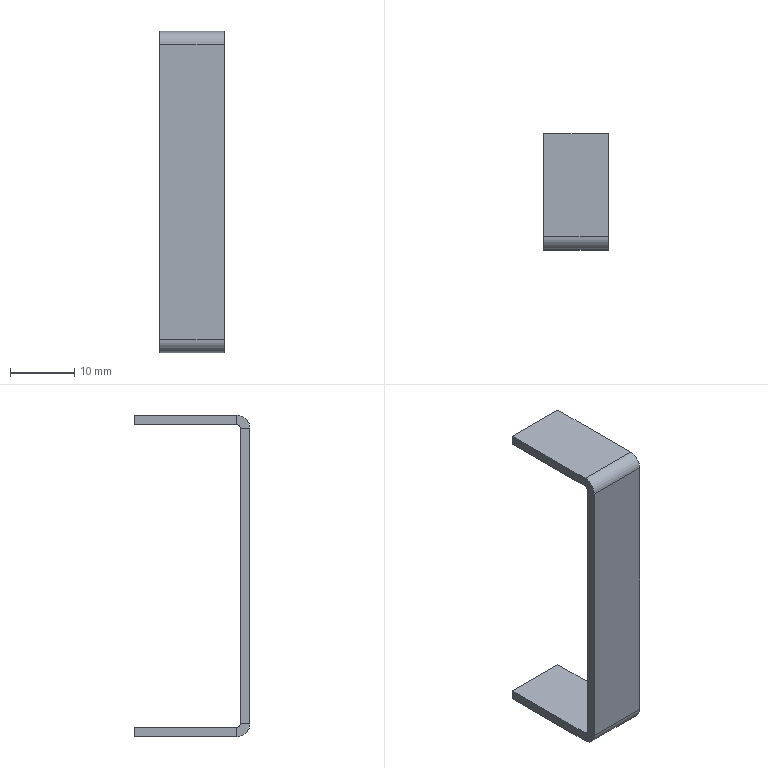Component | SolidWorks | OuterDoorAssembly1-1_CableSupportBracket-1 | 1 solid | 22 faces | box 10.01 x 18 x 50 mm | volume 1229 mm3 | plane 18 | cylinder 4 | commonest cylinder face diameters 4 x2 1 x2
STEP:
#1=CARTESIAN_POINT('',(17.943,6.43,12.714));
#2=VERTEX_POINT('',#1);
#3=CARTESIAN_POINT('',(17.943,6.489,12.714));
#4=VERTEX_POINT('',#3);
#5=CARTESIAN_POINT('',(17.943,6.43,12.714));
#6=DIRECTION('',(0.0003491,1.,-0.));
#7=VECTOR('',#6,39.37);
#8=LINE('',#5,#7);
#9=EDGE_CURVE('',#2,#4,#8,.T.);
#10=ORIENTED_EDGE('',*,*,#9,.F.);
#11=CARTESIAN_POINT('',(17.943,6.509,12.793));
#12=VERTEX_POINT('',#11);
#13=CARTESIAN_POINT('',(17.943,6.509,12.714));
#14=DIRECTION('',(1.,-0.0003491,0.));
#15=DIRECTION('',(-0.0003491,-1.,0.));
#16=AXIS2_PLACEMENT_3D('',#13,#14,#15);
#17=CIRCLE('',#16,0.07874);
#18=EDGE_CURVE('',#12,#2,#17,.T.);
#19=ORIENTED_EDGE('',*,*,#18,.F.);
#20=CARTESIAN_POINT('',(17.943,6.509,12.734));
#21=VERTEX_POINT('',#20);
#22=CARTESIAN_POINT('',(17.943,6.509,12.734));
#23=DIRECTION('',(-0.,0.,1.));
#24=VECTOR('',#23,39.37);
#25=LINE('',#22,#24);
#26=EDGE_CURVE('',#21,#12,#25,.T.);
#27=ORIENTED_EDGE('',*,*,#26,.F.);
#28=CARTESIAN_POINT('',(17.943,6.509,12.714));
#29=DIRECTION('',(1.,-0.0003491,0.));
#30=DIRECTION('',(-0.0003491,-1.,0.));
#31=AXIS2_PLACEMENT_3D('',#28,#29,#30);
#32=CIRCLE('',#31,0.01969);
#33=EDGE_CURVE('',#21,#4,#32,.T.);
#34=ORIENTED_EDGE('',*,*,#33,.T.);
#35=EDGE_LOOP('',(#10,#19,#27,#34));
#36=FACE_OUTER_BOUND('',#35,.T.);
#37=CARTESIAN_POINT('',(17.943,6.43,12.714));
#38=DIRECTION('',(-1.,0.0003491,-0.));
#39=DIRECTION('',(-0.0003491,-1.,0.));
#40=AXIS2_PLACEMENT_3D('',#37,#38,#39);
#41=PLANE('',#40);
#42=ADVANCED_FACE('',(#36),#41,.T.);
#43=CARTESIAN_POINT('',(17.943,6.43,10.903));
#44=VERTEX_POINT('',#43);
#45=CARTESIAN_POINT('',(17.943,6.43,12.793));
#46=DIRECTION('',(0.,-0.,-1.));
#47=VECTOR('',#46,39.37);
#48=LINE('',#45,#47);
#49=EDGE_CURVE('',#2,#44,#48,.T.);
#50=ORIENTED_EDGE('',*,*,#49,.F.);
#51=ORIENTED_EDGE('',*,*,#9,.T.);
#52=CARTESIAN_POINT('',(17.943,6.489,10.903));
#53=VERTEX_POINT('',#52);
#54=CARTESIAN_POINT('',(17.943,6.489,12.793));
#55=DIRECTION('',(0.,-0.,-1.));
#56=VECTOR('',#55,39.37);
#57=LINE('',#54,#56);
#58=EDGE_CURVE('',#4,#53,#57,.T.);
#59=ORIENTED_EDGE('',*,*,#58,.T.);
#60=CARTESIAN_POINT('',(17.943,6.489,10.903));
#61=DIRECTION('',(-0.0003491,-1.,0.));
#62=VECTOR('',#61,39.37);
#63=LINE('',#60,#62);
#64=EDGE_CURVE('',#53,#44,#63,.T.);
#65=ORIENTED_EDGE('',*,*,#64,.T.);
#66=EDGE_LOOP('',(#50,#51,#59,#65));
#67=FACE_OUTER_BOUND('',#66,.T.);
#68=CARTESIAN_POINT('',(17.943,6.509,12.734));
#69=DIRECTION('',(-1.,0.0003491,-0.));
#70=DIRECTION('',(-0.0003491,-1.,0.));
#71=AXIS2_PLACEMENT_3D('',#68,#69,#70);
#72=PLANE('',#71);
#73=ADVANCED_FACE('',(#67),#72,.T.);
#74=CARTESIAN_POINT('',(18.337,6.509,12.793));
#75=VERTEX_POINT('',#74);
#76=CARTESIAN_POINT('',(18.337,6.509,12.734));
#77=VERTEX_POINT('',#76);
#78=CARTESIAN_POINT('',(18.337,6.509,12.793));
#79=DIRECTION('',(0.,-0.,-1.));
#80=VECTOR('',#79,39.37);
#81=LINE('',#78,#80);
#82=EDGE_CURVE('',#75,#77,#81,.T.);
#83=ORIENTED_EDGE('',*,*,#82,.F.);
#84=CARTESIAN_POINT('',(18.337,6.43,12.714));
#85=VERTEX_POINT('',#84);
#86=CARTESIAN_POINT('',(18.337,6.509,12.714));
#87=DIRECTION('',(1.,-0.0003491,0.));
#88=DIRECTION('',(-0.0003491,-1.,0.));
#89=AXIS2_PLACEMENT_3D('',#86,#87,#88);
#90=CIRCLE('',#89,0.07874);
#91=EDGE_CURVE('',#75,#85,#90,.T.);
#92=ORIENTED_EDGE('',*,*,#91,.T.);
#93=CARTESIAN_POINT('',(18.337,6.489,12.714));
#94=VERTEX_POINT('',#93);
#95=CARTESIAN_POINT('',(18.337,6.489,12.714));
#96=DIRECTION('',(-0.0003491,-1.,0.));
#97=VECTOR('',#96,39.37);
#98=LINE('',#95,#97);
#99=EDGE_CURVE('',#94,#85,#98,.T.);
#100=ORIENTED_EDGE('',*,*,#99,.F.);
#101=CARTESIAN_POINT('',(18.337,6.509,12.714));
#102=DIRECTION('',(1.,-0.0003491,0.));
#103=DIRECTION('',(-0.0003491,-1.,0.));
#104=AXIS2_PLACEMENT_3D('',#101,#102,#103);
#105=CIRCLE('',#104,0.01969);
#106=EDGE_CURVE('',#77,#94,#105,.T.);
#107=ORIENTED_EDGE('',*,*,#106,.F.);
#108=EDGE_LOOP('',(#83,#92,#100,#107));
#109=FACE_OUTER_BOUND('',#108,.T.);
#110=CARTESIAN_POINT('',(18.337,6.509,12.793));
#111=DIRECTION('',(1.,-0.0003491,0.));
#112=DIRECTION('',(0.0003491,1.,-0.));
#113=AXIS2_PLACEMENT_3D('',#110,#111,#112);
#114=PLANE('',#113);
#115=ADVANCED_FACE('',(#109),#114,.T.);
#116=CARTESIAN_POINT('',(18.337,7.139,12.793));
#117=VERTEX_POINT('',#116);
#118=CARTESIAN_POINT('',(18.337,7.139,12.793));
#119=DIRECTION('',(-0.0003491,-1.,0.));
#120=VECTOR('',#119,39.37);
#121=LINE('',#118,#120);
#122=EDGE_CURVE('',#117,#75,#121,.T.);
#123=ORIENTED_EDGE('',*,*,#122,.T.);
#124=ORIENTED_EDGE('',*,*,#82,.T.);
#125=CARTESIAN_POINT('',(18.337,7.139,12.734));
#126=VERTEX_POINT('',#125);
#127=CARTESIAN_POINT('',(18.337,7.139,12.734));
#128=DIRECTION('',(-0.0003491,-1.,0.));
#129=VECTOR('',#128,39.37);
#130=LINE('',#127,#129);
#131=EDGE_CURVE('',#126,#77,#130,.T.);
#132=ORIENTED_EDGE('',*,*,#131,.F.);
#133=CARTESIAN_POINT('',(18.337,7.139,12.734));
#134=DIRECTION('',(-0.,0.,1.));
#135=VECTOR('',#134,39.37);
#136=LINE('',#133,#135);
#137=EDGE_CURVE('',#126,#117,#136,.T.);
#138=ORIENTED_EDGE('',*,*,#137,.T.);
#139=EDGE_LOOP('',(#123,#124,#132,#138));
#140=FACE_OUTER_BOUND('',#139,.T.);
#141=CARTESIAN_POINT('',(18.337,6.489,12.714));
#142=DIRECTION('',(1.,-0.0003491,0.));
#143=DIRECTION('',(0.0003491,1.,-0.));
#144=AXIS2_PLACEMENT_3D('',#141,#142,#143);
#145=PLANE('',#144);
#146=ADVANCED_FACE('',(#140),#145,.T.);
#147=CARTESIAN_POINT('',(17.943,6.509,10.824));
#148=VERTEX_POINT('',#147);
#149=CARTESIAN_POINT('',(17.943,6.509,10.883));
#150=VERTEX_POINT('',#149);
#151=CARTESIAN_POINT('',(17.943,6.509,10.824));
#152=DIRECTION('',(-0.,0.,1.));
#153=VECTOR('',#152,39.37);
#154=LINE('',#151,#153);
#155=EDGE_CURVE('',#148,#150,#154,.T.);
#156=ORIENTED_EDGE('',*,*,#155,.F.);
#157=CARTESIAN_POINT('',(17.943,6.509,10.903));
#158=DIRECTION('',(1.,-0.0003491,0.));
#159=DIRECTION('',(-0.0003491,-1.,0.));
#160=AXIS2_PLACEMENT_3D('',#157,#158,#159);
#161=CIRCLE('',#160,0.07874);
#162=EDGE_CURVE('',#44,#148,#161,.T.);
#163=ORIENTED_EDGE('',*,*,#162,.F.);
#164=ORIENTED_EDGE('',*,*,#64,.F.);
#165=CARTESIAN_POINT('',(17.943,6.509,10.903));
#166=DIRECTION('',(1.,-0.0003491,0.));
#167=DIRECTION('',(-0.0003491,-1.,0.));
#168=AXIS2_PLACEMENT_3D('',#165,#166,#167);
#169=CIRCLE('',#168,0.01969);
#170=EDGE_CURVE('',#53,#150,#169,.T.);
#171=ORIENTED_EDGE('',*,*,#170,.T.);
#172=EDGE_LOOP('',(#156,#163,#164,#171));
#173=FACE_OUTER_BOUND('',#172,.T.);
#174=CARTESIAN_POINT('',(17.943,6.509,10.824));
#175=DIRECTION('',(-1.,0.0003491,-0.));
#176=DIRECTION('',(-0.0003491,-1.,0.));
#177=AXIS2_PLACEMENT_3D('',#174,#175,#176);
#178=PLANE('',#177);
#179=ADVANCED_FACE('',(#173),#178,.T.);
#180=CARTESIAN_POINT('',(17.944,7.139,10.824));
#181=VERTEX_POINT('',#180);
#182=CARTESIAN_POINT('',(17.943,6.43,10.824));
#183=DIRECTION('',(0.0003491,1.,-0.));
#184=VECTOR('',#183,39.37);
#185=LINE('',#182,#184);
#186=EDGE_CURVE('',#148,#181,#185,.T.);
#187=ORIENTED_EDGE('',*,*,#186,.F.);
#188=ORIENTED_EDGE('',*,*,#155,.T.);
#189=CARTESIAN_POINT('',(17.944,7.139,10.883));
#190=VERTEX_POINT('',#189);
#191=CARTESIAN_POINT('',(17.943,6.43,10.883));
#192=DIRECTION('',(0.0003491,1.,-0.));
#193=VECTOR('',#192,39.37);
#194=LINE('',#191,#193);
#195=EDGE_CURVE('',#150,#190,#194,.T.);
#196=ORIENTED_EDGE('',*,*,#195,.T.);
#197=CARTESIAN_POINT('',(17.944,7.139,10.824));
#198=DIRECTION('',(-0.,0.,1.));
#199=VECTOR('',#198,39.37);
#200=LINE('',#197,#199);
#201=EDGE_CURVE('',#181,#190,#200,.T.);
#202=ORIENTED_EDGE('',*,*,#201,.F.);
#203=EDGE_LOOP('',(#187,#188,#196,#202));
#204=FACE_OUTER_BOUND('',#203,.T.);
#205=CARTESIAN_POINT('',(17.943,6.489,10.903));
#206=DIRECTION('',(-1.,0.0003491,-0.));
#207=DIRECTION('',(-0.0003491,-1.,0.));
#208=AXIS2_PLACEMENT_3D('',#205,#206,#207);
#209=PLANE('',#208);
#210=ADVANCED_FACE('',(#204),#209,.T.);
#211=CARTESIAN_POINT('',(18.337,6.43,10.903));
#212=VERTEX_POINT('',#211);
#213=CARTESIAN_POINT('',(18.337,6.489,10.903));
#214=VERTEX_POINT('',#213);
#215=CARTESIAN_POINT('',(18.337,6.43,10.903));
#216=DIRECTION('',(0.0003491,1.,-0.));
#217=VECTOR('',#216,39.37);
#218=LINE('',#215,#217);
#219=EDGE_CURVE('',#212,#214,#218,.T.);
#220=ORIENTED_EDGE('',*,*,#219,.F.);
#221=CARTESIAN_POINT('',(18.337,6.509,10.824));
#222=VERTEX_POINT('',#221);
#223=CARTESIAN_POINT('',(18.337,6.509,10.903));
#224=DIRECTION('',(1.,-0.0003491,0.));
#225=DIRECTION('',(-0.0003491,-1.,0.));
#226=AXIS2_PLACEMENT_3D('',#223,#224,#225);
#227=CIRCLE('',#226,0.07874);
#228=EDGE_CURVE('',#212,#222,#227,.T.);
#229=ORIENTED_EDGE('',*,*,#228,.T.);
#230=CARTESIAN_POINT('',(18.337,6.509,10.883));
#231=VERTEX_POINT('',#230);
#232=CARTESIAN_POINT('',(18.337,6.509,10.883));
#233=DIRECTION('',(0.,-0.,-1.));
#234=VECTOR('',#233,39.37);
#235=LINE('',#232,#234);
#236=EDGE_CURVE('',#231,#222,#235,.T.);
#237=ORIENTED_EDGE('',*,*,#236,.F.);
#238=CARTESIAN_POINT('',(18.337,6.509,10.903));
#239=DIRECTION('',(1.,-0.0003491,0.));
#240=DIRECTION('',(-0.0003491,-1.,0.));
#241=AXIS2_PLACEMENT_3D('',#238,#239,#240);
#242=CIRCLE('',#241,0.01969);
#243=EDGE_CURVE('',#214,#231,#242,.T.);
#244=ORIENTED_EDGE('',*,*,#243,.F.);
#245=EDGE_LOOP('',(#220,#229,#237,#244));
#246=FACE_OUTER_BOUND('',#245,.T.);
#247=CARTESIAN_POINT('',(18.337,6.43,10.903));
#248=DIRECTION('',(1.,-0.0003491,0.));
#249=DIRECTION('',(0.0003491,1.,-0.));
#250=AXIS2_PLACEMENT_3D('',#247,#248,#249);
#251=PLANE('',#250);
#252=ADVANCED_FACE('',(#246),#251,.T.);
#253=CARTESIAN_POINT('',(18.337,6.43,12.793));
#254=DIRECTION('',(0.,-0.,-1.));
#255=VECTOR('',#254,39.37);
#256=LINE('',#253,#255);
#257=EDGE_CURVE('',#85,#212,#256,.T.);
#258=ORIENTED_EDGE('',*,*,#257,.T.);
#259=ORIENTED_EDGE('',*,*,#219,.T.);
#260=CARTESIAN_POINT('',(18.337,6.489,12.793));
#261=DIRECTION('',(0.,-0.,-1.));
#262=VECTOR('',#261,39.37);
#263=LINE('',#260,#262);
#264=EDGE_CURVE('',#94,#214,#263,.T.);
#265=ORIENTED_EDGE('',*,*,#264,.F.);
#266=ORIENTED_EDGE('',*,*,#99,.T.);
#267=EDGE_LOOP('',(#258,#259,#265,#266));
#268=FACE_OUTER_BOUND('',#267,.T.);
#269=CARTESIAN_POINT('',(18.337,6.509,10.883));
#270=DIRECTION('',(1.,-0.0003491,0.));
#271=DIRECTION('',(0.0003491,1.,-0.));
#272=AXIS2_PLACEMENT_3D('',#269,#270,#271);
#273=PLANE('',#272);
#274=ADVANCED_FACE('',(#268),#273,.T.);
#275=CARTESIAN_POINT('',(18.337,7.139,10.883));
#276=VERTEX_POINT('',#275);
#277=CARTESIAN_POINT('',(18.337,6.43,10.883));
#278=DIRECTION('',(0.0003491,1.,-0.));
#279=VECTOR('',#278,39.37);
#280=LINE('',#277,#279);
#281=EDGE_CURVE('',#231,#276,#280,.T.);
#282=ORIENTED_EDGE('',*,*,#281,.T.);
#283=CARTESIAN_POINT('',(17.944,7.139,10.883));
#284=DIRECTION('',(1.,-0.0003491,0.));
#285=VECTOR('',#284,39.37);
#286=LINE('',#283,#285);
#287=EDGE_CURVE('',#190,#276,#286,.T.);
#288=ORIENTED_EDGE('',*,*,#287,.F.);
#289=ORIENTED_EDGE('',*,*,#195,.F.);
#290=CARTESIAN_POINT('',(17.943,6.509,10.883));
#291=DIRECTION('',(1.,-0.0003491,0.));
#292=VECTOR('',#291,39.37);
#293=LINE('',#290,#292);
#294=EDGE_CURVE('',#150,#231,#293,.T.);
#295=ORIENTED_EDGE('',*,*,#294,.T.);
#296=EDGE_LOOP('',(#282,#288,#289,#295));
#297=FACE_OUTER_BOUND('',#296,.T.);
#298=CARTESIAN_POINT('',(17.943,6.43,10.883));
#299=DIRECTION('',(0.,-0.,-1.));
#300=DIRECTION('',(1.,-0.0003491,0.));
#301=AXIS2_PLACEMENT_3D('',#298,#299,#300);
#302=PLANE('',#301);
#303=ADVANCED_FACE('',(#297),#302,.F.);
#304=CARTESIAN_POINT('',(18.337,7.139,10.824));
#305=VERTEX_POINT('',#304);
#306=CARTESIAN_POINT('',(18.337,7.139,10.824));
#307=DIRECTION('',(-0.,0.,1.));
#308=VECTOR('',#307,39.37);
#309=LINE('',#306,#308);
#310=EDGE_CURVE('',#305,#276,#309,.T.);
#311=ORIENTED_EDGE('',*,*,#310,.F.);
#312=CARTESIAN_POINT('',(17.944,7.139,10.824));
#313=DIRECTION('',(1.,-0.0003491,0.));
#314=VECTOR('',#313,39.37);
#315=LINE('',#312,#314);
#316=EDGE_CURVE('',#181,#305,#315,.T.);
#317=ORIENTED_EDGE('',*,*,#316,.F.);
#318=ORIENTED_EDGE('',*,*,#201,.T.);
#319=ORIENTED_EDGE('',*,*,#287,.T.);
#320=EDGE_LOOP('',(#311,#317,#318,#319));
#321=FACE_OUTER_BOUND('',#320,.T.);
#322=CARTESIAN_POINT('',(17.944,7.139,10.824));
#323=DIRECTION('',(0.0003491,1.,-0.));
#324=DIRECTION('',(-1.,0.0003491,-0.));
#325=AXIS2_PLACEMENT_3D('',#322,#323,#324);
#326=PLANE('',#325);
#327=ADVANCED_FACE('',(#321),#326,.T.);
#328=CARTESIAN_POINT('',(18.337,6.43,10.824));
#329=DIRECTION('',(0.0003491,1.,-0.));
#330=VECTOR('',#329,39.37);
#331=LINE('',#328,#330);
#332=EDGE_CURVE('',#222,#305,#331,.T.);
#333=ORIENTED_EDGE('',*,*,#332,.F.);
#334=CARTESIAN_POINT('',(17.943,6.509,10.824));
#335=DIRECTION('',(1.,-0.0003491,0.));
#336=VECTOR('',#335,39.37);
#337=LINE('',#334,#336);
#338=EDGE_CURVE('',#148,#222,#337,.T.);
#339=ORIENTED_EDGE('',*,*,#338,.F.);
#340=ORIENTED_EDGE('',*,*,#186,.T.);
#341=ORIENTED_EDGE('',*,*,#316,.T.);
#342=EDGE_LOOP('',(#333,#339,#340,#341));
#343=FACE_OUTER_BOUND('',#342,.T.);
#344=CARTESIAN_POINT('',(17.943,6.43,10.824));
#345=DIRECTION('',(0.,-0.,-1.));
#346=DIRECTION('',(1.,-0.0003491,0.));
#347=AXIS2_PLACEMENT_3D('',#344,#345,#346);
#348=PLANE('',#347);
#349=ADVANCED_FACE('',(#343),#348,.T.);
#350=ORIENTED_EDGE('',*,*,#228,.F.);
#351=CARTESIAN_POINT('',(17.943,6.43,10.903));
#352=DIRECTION('',(1.,-0.0003491,0.));
#353=VECTOR('',#352,39.37);
#354=LINE('',#351,#353);
#355=EDGE_CURVE('',#44,#212,#354,.T.);
#356=ORIENTED_EDGE('',*,*,#355,.F.);
#357=ORIENTED_EDGE('',*,*,#162,.T.);
#358=ORIENTED_EDGE('',*,*,#338,.T.);
#359=EDGE_LOOP('',(#350,#356,#357,#358));
#360=FACE_OUTER_BOUND('',#359,.T.);
#361=CARTESIAN_POINT('',(17.943,6.509,10.903));
#362=DIRECTION('',(1.,-0.0003491,0.));
#363=DIRECTION('',(0.0003491,1.,0.));
#364=AXIS2_PLACEMENT_3D('',#361,#362,#363);
#365=CYLINDRICAL_SURFACE('',#364,0.07874);
#366=ADVANCED_FACE('',(#360),#365,.T.);
#367=ORIENTED_EDGE('',*,*,#257,.F.);
#368=CARTESIAN_POINT('',(17.943,6.43,12.714));
#369=DIRECTION('',(1.,-0.0003491,0.));
#370=VECTOR('',#369,39.37);
#371=LINE('',#368,#370);
#372=EDGE_CURVE('',#2,#85,#371,.T.);
#373=ORIENTED_EDGE('',*,*,#372,.F.);
#374=ORIENTED_EDGE('',*,*,#49,.T.);
#375=ORIENTED_EDGE('',*,*,#355,.T.);
#376=EDGE_LOOP('',(#367,#373,#374,#375));
#377=FACE_OUTER_BOUND('',#376,.T.);
#378=CARTESIAN_POINT('',(17.943,6.43,12.793));
#379=DIRECTION('',(-0.0003491,-1.,0.));
#380=DIRECTION('',(-0.,0.,1.));
#381=AXIS2_PLACEMENT_3D('',#378,#379,#380);
#382=PLANE('',#381);
#383=ADVANCED_FACE('',(#377),#382,.T.);
#384=ORIENTED_EDGE('',*,*,#91,.F.);
#385=CARTESIAN_POINT('',(17.943,6.509,12.793));
#386=DIRECTION('',(1.,-0.0003491,0.));
#387=VECTOR('',#386,39.37);
#388=LINE('',#385,#387);
#389=EDGE_CURVE('',#12,#75,#388,.T.);
#390=ORIENTED_EDGE('',*,*,#389,.F.);
#391=ORIENTED_EDGE('',*,*,#18,.T.);
#392=ORIENTED_EDGE('',*,*,#372,.T.);
#393=EDGE_LOOP('',(#384,#390,#391,#392));
#394=FACE_OUTER_BOUND('',#393,.T.);
#395=CARTESIAN_POINT('',(17.943,6.509,12.714));
#396=DIRECTION('',(1.,-0.0003491,0.));
#397=DIRECTION('',(0.0003491,1.,0.));
#398=AXIS2_PLACEMENT_3D('',#395,#396,#397);
#399=CYLINDRICAL_SURFACE('',#398,0.07874);
#400=ADVANCED_FACE('',(#394),#399,.T.);
#401=ORIENTED_EDGE('',*,*,#122,.F.);
#402=CARTESIAN_POINT('',(17.944,7.139,12.793));
#403=VERTEX_POINT('',#402);
#404=CARTESIAN_POINT('',(17.944,7.139,12.793));
#405=DIRECTION('',(1.,-0.0003491,0.));
#406=VECTOR('',#405,39.37);
#407=LINE('',#404,#406);
#408=EDGE_CURVE('',#403,#117,#407,.T.);
#409=ORIENTED_EDGE('',*,*,#408,.F.);
#410=CARTESIAN_POINT('',(17.944,7.139,12.793));
#411=DIRECTION('',(-0.0003491,-1.,0.));
#412=VECTOR('',#411,39.37);
#413=LINE('',#410,#412);
#414=EDGE_CURVE('',#403,#12,#413,.T.);
#415=ORIENTED_EDGE('',*,*,#414,.T.);
#416=ORIENTED_EDGE('',*,*,#389,.T.);
#417=EDGE_LOOP('',(#401,#409,#415,#416));
#418=FACE_OUTER_BOUND('',#417,.T.);
#419=CARTESIAN_POINT('',(17.944,7.139,12.793));
#420=DIRECTION('',(-0.,0.,1.));
#421=DIRECTION('',(-1.,0.0003491,-0.));
#422=AXIS2_PLACEMENT_3D('',#419,#420,#421);
#423=PLANE('',#422);
#424=ADVANCED_FACE('',(#418),#423,.T.);
#425=ORIENTED_EDGE('',*,*,#137,.F.);
#426=CARTESIAN_POINT('',(17.944,7.139,12.734));
#427=VERTEX_POINT('',#426);
#428=CARTESIAN_POINT('',(17.944,7.139,12.734));
#429=DIRECTION('',(1.,-0.0003491,0.));
#430=VECTOR('',#429,39.37);
#431=LINE('',#428,#430);
#432=EDGE_CURVE('',#427,#126,#431,.T.);
#433=ORIENTED_EDGE('',*,*,#432,.F.);
#434=CARTESIAN_POINT('',(17.944,7.139,12.734));
#435=DIRECTION('',(-0.,0.,1.));
#436=VECTOR('',#435,39.37);
#437=LINE('',#434,#436);
#438=EDGE_CURVE('',#427,#403,#437,.T.);
#439=ORIENTED_EDGE('',*,*,#438,.T.);
#440=ORIENTED_EDGE('',*,*,#408,.T.);
#441=EDGE_LOOP('',(#425,#433,#439,#440));
#442=FACE_OUTER_BOUND('',#441,.T.);
#443=CARTESIAN_POINT('',(17.944,7.139,12.734));
#444=DIRECTION('',(0.0003491,1.,-0.));
#445=DIRECTION('',(-1.,0.0003491,-0.));
#446=AXIS2_PLACEMENT_3D('',#443,#444,#445);
#447=PLANE('',#446);
#448=ADVANCED_FACE('',(#442),#447,.T.);
#449=ORIENTED_EDGE('',*,*,#131,.T.);
#450=CARTESIAN_POINT('',(17.943,6.509,12.734));
#451=DIRECTION('',(1.,-0.0003491,0.));
#452=VECTOR('',#451,39.37);
#453=LINE('',#450,#452);
#454=EDGE_CURVE('',#21,#77,#453,.T.);
#455=ORIENTED_EDGE('',*,*,#454,.F.);
#456=CARTESIAN_POINT('',(17.944,7.139,12.734));
#457=DIRECTION('',(-0.0003491,-1.,0.));
#458=VECTOR('',#457,39.37);
#459=LINE('',#456,#458);
#460=EDGE_CURVE('',#427,#21,#459,.T.);
#461=ORIENTED_EDGE('',*,*,#460,.F.);
#462=ORIENTED_EDGE('',*,*,#432,.T.);
#463=EDGE_LOOP('',(#449,#455,#461,#462));
#464=FACE_OUTER_BOUND('',#463,.T.);
#465=CARTESIAN_POINT('',(17.944,7.139,12.734));
#466=DIRECTION('',(-0.,0.,1.));
#467=DIRECTION('',(-1.,0.0003491,-0.));
#468=AXIS2_PLACEMENT_3D('',#465,#466,#467);
#469=PLANE('',#468);
#470=ADVANCED_FACE('',(#464),#469,.F.);
#471=ORIENTED_EDGE('',*,*,#106,.T.);
#472=CARTESIAN_POINT('',(17.943,6.489,12.714));
#473=DIRECTION('',(1.,-0.0003491,0.));
#474=VECTOR('',#473,39.37);
#475=LINE('',#472,#474);
#476=EDGE_CURVE('',#4,#94,#475,.T.);
#477=ORIENTED_EDGE('',*,*,#476,.F.);
#478=ORIENTED_EDGE('',*,*,#33,.F.);
#479=ORIENTED_EDGE('',*,*,#454,.T.);
#480=EDGE_LOOP('',(#471,#477,#478,#479));
#481=FACE_OUTER_BOUND('',#480,.T.);
#482=CARTESIAN_POINT('',(17.943,6.509,12.714));
#483=DIRECTION('',(1.,-0.0003491,0.));
#484=DIRECTION('',(0.0003491,1.,0.));
#485=AXIS2_PLACEMENT_3D('',#482,#483,#484);
#486=CYLINDRICAL_SURFACE('',#485,0.01969);
#487=ADVANCED_FACE('',(#481),#486,.F.);
#488=ORIENTED_EDGE('',*,*,#264,.T.);
#489=CARTESIAN_POINT('',(17.943,6.489,10.903));
#490=DIRECTION('',(1.,-0.0003491,0.));
#491=VECTOR('',#490,39.37);
#492=LINE('',#489,#491);
#493=EDGE_CURVE('',#53,#214,#492,.T.);
#494=ORIENTED_EDGE('',*,*,#493,.F.);
#495=ORIENTED_EDGE('',*,*,#58,.F.);
#496=ORIENTED_EDGE('',*,*,#476,.T.);
#497=EDGE_LOOP('',(#488,#494,#495,#496));
#498=FACE_OUTER_BOUND('',#497,.T.);
#499=CARTESIAN_POINT('',(17.943,6.489,12.793));
#500=DIRECTION('',(-0.0003491,-1.,0.));
#501=DIRECTION('',(-0.,0.,1.));
#502=AXIS2_PLACEMENT_3D('',#499,#500,#501);
#503=PLANE('',#502);
#504=ADVANCED_FACE('',(#498),#503,.F.);
#505=ORIENTED_EDGE('',*,*,#243,.T.);
#506=ORIENTED_EDGE('',*,*,#294,.F.);
#507=ORIENTED_EDGE('',*,*,#170,.F.);
#508=ORIENTED_EDGE('',*,*,#493,.T.);
#509=EDGE_LOOP('',(#505,#506,#507,#508));
#510=FACE_OUTER_BOUND('',#509,.T.);
#511=CARTESIAN_POINT('',(17.943,6.509,10.903));
#512=DIRECTION('',(1.,-0.0003491,0.));
#513=DIRECTION('',(0.0003491,1.,0.));
#514=AXIS2_PLACEMENT_3D('',#511,#512,#513);
#515=CYLINDRICAL_SURFACE('',#514,0.01969);
#516=ADVANCED_FACE('',(#510),#515,.F.);
#517=ORIENTED_EDGE('',*,*,#460,.T.);
#518=ORIENTED_EDGE('',*,*,#26,.T.);
#519=ORIENTED_EDGE('',*,*,#414,.F.);
#520=ORIENTED_EDGE('',*,*,#438,.F.);
#521=EDGE_LOOP('',(#517,#518,#519,#520));
#522=FACE_OUTER_BOUND('',#521,.T.);
#523=CARTESIAN_POINT('',(17.943,6.509,10.903));
#524=DIRECTION('',(-1.,0.0003491,-0.));
#525=DIRECTION('',(-0.0003491,-1.,0.));
#526=AXIS2_PLACEMENT_3D('',#523,#524,#525);
#527=PLANE('',#526);
#528=ADVANCED_FACE('',(#522),#527,.T.);
#529=ORIENTED_EDGE('',*,*,#281,.F.);
#530=ORIENTED_EDGE('',*,*,#236,.T.);
#531=ORIENTED_EDGE('',*,*,#332,.T.);
#532=ORIENTED_EDGE('',*,*,#310,.T.);
#533=EDGE_LOOP('',(#529,#530,#531,#532));
#534=FACE_OUTER_BOUND('',#533,.T.);
#535=CARTESIAN_POINT('',(18.337,6.509,10.903));
#536=DIRECTION('',(-1.,0.0003491,-0.));
#537=DIRECTION('',(-0.0003491,-1.,0.));
#538=AXIS2_PLACEMENT_3D('',#535,#536,#537);
#539=PLANE('',#538);
#540=ADVANCED_FACE('',(#534),#539,.F.);
#541=CLOSED_SHELL('',(#42,#73,#115,#146,#179,#210,#252,#274,#303,#327,#349,#366,#383,#400,#424,#448,#470,#487,#504,#516,#528,#540));
#542=MANIFOLD_SOLID_BREP('',#541);
#543=CARTESIAN_POINT('',(0.,0.,0.));
#544=DIRECTION('',(0.,0.,1.));
#545=DIRECTION('',(1.,0.,0.));
#546=AXIS2_PLACEMENT_3D('',#543,#544,#545);
#547=(LENGTH_UNIT()NAMED_UNIT(*)SI_UNIT($,.METRE.));
#548=LENGTH_MEASURE_WITH_UNIT(LENGTH_MEASURE(0.0254),#547);
#549=DIMENSIONAL_EXPONENTS(1.,0.,0.,0.,0.,0.,0.);
#550=(CONVERSION_BASED_UNIT('',#548)LENGTH_UNIT()NAMED_UNIT(#549));
#551=UNCERTAINTY_MEASURE_WITH_UNIT(LENGTH_MEASURE(0.00001),#550,'','');
#552=(NAMED_UNIT(*)PLANE_ANGLE_UNIT()SI_UNIT($,.RADIAN.));
#553=(NAMED_UNIT(*)SI_UNIT($,.STERADIAN.)SOLID_ANGLE_UNIT());
#554=(GEOMETRIC_REPRESENTATION_CONTEXT(3)GLOBAL_UNCERTAINTY_ASSIGNED_CONTEXT((#551))GLOBAL_UNIT_ASSIGNED_CONTEXT((#550,#552,#553))REPRESENTATION_CONTEXT('',''));
#555=ADVANCED_BREP_SHAPE_REPRESENTATION('',(#542,#546),#554);
#556=COLOUR_RGB('',0.7922,0.8196,0.9333);
#557=FILL_AREA_STYLE_COLOUR('',#556);
#558=FILL_AREA_STYLE('',(#557));
#559=SURFACE_STYLE_FILL_AREA(#558);
#560=SURFACE_SIDE_STYLE('',(#559));
#561=SURFACE_STYLE_USAGE(.BOTH.,#560);
#562=PRESENTATION_STYLE_ASSIGNMENT((#561));
#563=STYLED_ITEM('',(#562),#542);
#564=(LENGTH_UNIT()NAMED_UNIT(*)SI_UNIT($,.METRE.));
#565=LENGTH_MEASURE_WITH_UNIT(LENGTH_MEASURE(0.0254),#564);
#566=DIMENSIONAL_EXPONENTS(1.,0.,0.,0.,0.,0.,0.);
#567=(CONVERSION_BASED_UNIT('',#565)LENGTH_UNIT()NAMED_UNIT(#566));
#568=UNCERTAINTY_MEASURE_WITH_UNIT(LENGTH_MEASURE(0.00001),#567,'','');
#569=(NAMED_UNIT(*)PLANE_ANGLE_UNIT()SI_UNIT($,.RADIAN.));
#570=(NAMED_UNIT(*)SI_UNIT($,.STERADIAN.)SOLID_ANGLE_UNIT());
#571=(GEOMETRIC_REPRESENTATION_CONTEXT(3)GLOBAL_UNCERTAINTY_ASSIGNED_CONTEXT((#568))GLOBAL_UNIT_ASSIGNED_CONTEXT((#567,#569,#570))REPRESENTATION_CONTEXT('',''));
#572=MECHANICAL_DESIGN_GEOMETRIC_PRESENTATION_REPRESENTATION('',(#563),#571);
#573=PRESENTATION_LAYER_ASSIGNMENT('','',(#563));